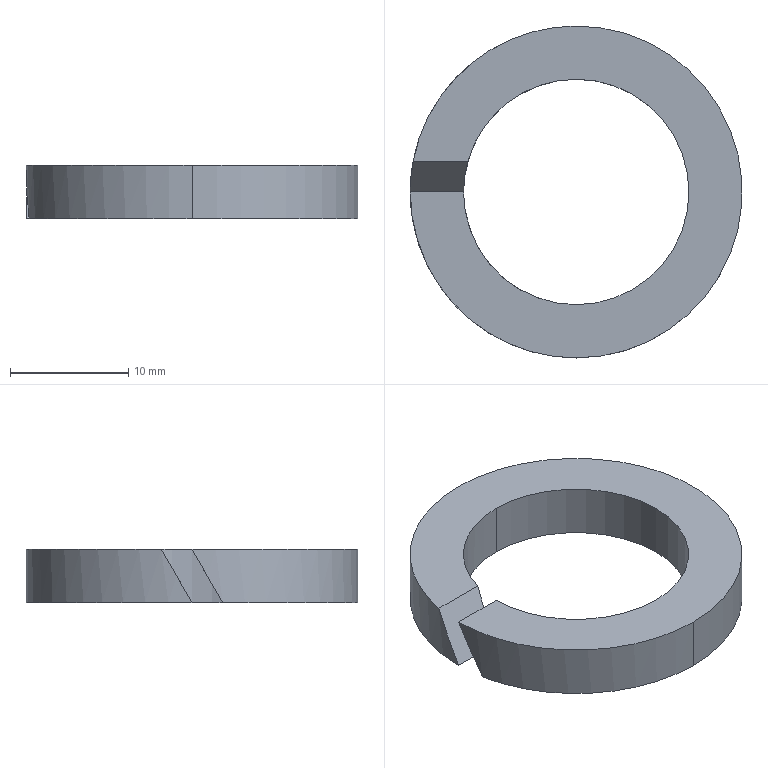Component | SolidWorks | Cylinder-1_spring lock washers--normal type gb-11 | 1 solid | 10 faces | box 28.04 x 28.04 x 4.5 mm | volume 1445 mm3 | cylinder 6 | plane 4 | commonest cylinder face diameters 19.04 x3 28.04 x3
build123d program:
from build123d import *

# Parameters (mm, degrees)
SKETCH1_R          = 14.02
SKETCH1_R_2        = 9.52
BASE_EXTRUDE_DEPTH = 4.5
CUT_EXTRUDE1_DEPTH = 21.332


with BuildPart() as part:
    # Sketch1 → Base-Extrude (new body)
    with BuildSketch(Plane.XY):
        Circle(SKETCH1_R)
        Circle(SKETCH1_R_2, mode=Mode.SUBTRACT)
    extrude(amount=-BASE_EXTRUDE_DEPTH)

    # Sketch2 → Cut-Extrude1 (cut, through all)
    with BuildSketch(Plane(origin=(0, 0, 0), x_dir=(1, 0, 0), z_dir=(0, 1, 0))):
        Polygon((0, 4.5), (2.598, 0), (0, 0), (-2.598, 4.5), align=None)
    extrude(amount=CUT_EXTRUDE1_DEPTH, mode=Mode.SUBTRACT)


solid = part.part

# Placed as in the assembly
solid = solid.moved(Location((-180.557, 26.412, -327.351), (0, 0, 90)))
STEP:
#1=COLOUR_RGB('',0.7922,0.8196,0.9333);
#2=FILL_AREA_STYLE_COLOUR('',#1);
#3=FILL_AREA_STYLE('',(#2));
#4=SURFACE_STYLE_FILL_AREA(#3);
#5=SURFACE_SIDE_STYLE('',(#4));
#6=SURFACE_STYLE_USAGE(.BOTH.,#5);
#7=PRESENTATION_STYLE_ASSIGNMENT((#6));
#8=CARTESIAN_POINT('',(-7.109,1.415,-12.888));
#9=VERTEX_POINT('',#8);
#10=CARTESIAN_POINT('',(-7.109,0.665,-12.888));
#11=VERTEX_POINT('',#10);
#12=CARTESIAN_POINT('',(-7.109,1.04,-12.888));
#13=DIRECTION('',(0.,-0.,-1.));
#14=DIRECTION('',(0.,-1.,0.));
#15=AXIS2_PLACEMENT_3D('',#12,#13,#14);
#16=CIRCLE('',#15,0.3748);
#17=EDGE_CURVE('',#9,#11,#16,.T.);
#18=ORIENTED_EDGE('',*,*,#17,.F.);
#19=CARTESIAN_POINT('',(-7.109,1.415,-13.065));
#20=VERTEX_POINT('',#19);
#21=CARTESIAN_POINT('',(-7.109,1.415,-12.888));
#22=DIRECTION('',(0.,-0.,-1.));
#23=VECTOR('',#22,39.37);
#24=LINE('',#21,#23);
#25=EDGE_CURVE('',#9,#20,#24,.T.);
#26=ORIENTED_EDGE('',*,*,#25,.T.);
#27=CARTESIAN_POINT('',(-7.109,0.665,-13.065));
#28=VERTEX_POINT('',#27);
#29=CARTESIAN_POINT('',(-7.109,1.04,-13.065));
#30=DIRECTION('',(0.,-0.,-1.));
#31=DIRECTION('',(0.,-1.,0.));
#32=AXIS2_PLACEMENT_3D('',#29,#30,#31);
#33=CIRCLE('',#32,0.3748);
#34=EDGE_CURVE('',#20,#28,#33,.T.);
#35=ORIENTED_EDGE('',*,*,#34,.T.);
#36=CARTESIAN_POINT('',(-7.109,0.665,-12.888));
#37=DIRECTION('',(0.,-0.,-1.));
#38=VECTOR('',#37,39.37);
#39=LINE('',#36,#38);
#40=EDGE_CURVE('',#11,#28,#39,.T.);
#41=ORIENTED_EDGE('',*,*,#40,.F.);
#42=EDGE_LOOP('',(#18,#26,#35,#41));
#43=FACE_OUTER_BOUND('',#42,.T.);
#44=CARTESIAN_POINT('',(-7.109,1.04,-12.888));
#45=DIRECTION('',(0.,-0.,-1.));
#46=DIRECTION('',(0.,-1.,0.));
#47=AXIS2_PLACEMENT_3D('',#44,#45,#46);
#48=CYLINDRICAL_SURFACE('',#47,0.3748);
#49=ADVANCED_FACE('',(#43),#48,.F.);
#50=CARTESIAN_POINT('',(-7.483,1.04,-12.888));
#51=VERTEX_POINT('',#50);
#52=CARTESIAN_POINT('',(-7.109,1.04,-12.888));
#53=DIRECTION('',(0.,-0.,-1.));
#54=DIRECTION('',(0.,-1.,0.));
#55=AXIS2_PLACEMENT_3D('',#52,#53,#54);
#56=CIRCLE('',#55,0.3748);
#57=EDGE_CURVE('',#11,#51,#56,.T.);
#58=ORIENTED_EDGE('',*,*,#57,.F.);
#59=ORIENTED_EDGE('',*,*,#40,.T.);
#60=CARTESIAN_POINT('',(-7.469,0.9376,-13.065));
#61=VERTEX_POINT('',#60);
#62=CARTESIAN_POINT('',(-7.109,1.04,-13.065));
#63=DIRECTION('',(0.,-0.,-1.));
#64=DIRECTION('',(0.,-1.,0.));
#65=AXIS2_PLACEMENT_3D('',#62,#63,#64);
#66=CIRCLE('',#65,0.3748);
#67=EDGE_CURVE('',#28,#61,#66,.T.);
#68=ORIENTED_EDGE('',*,*,#67,.T.);
#69=CARTESIAN_POINT('',(-7.483,1.04,-12.888));
#70=CARTESIAN_POINT('',(-7.483,1.005,-12.948));
#71=CARTESIAN_POINT('',(-7.479,0.9709,-13.007));
#72=CARTESIAN_POINT('',(-7.469,0.9376,-13.065));
#73=(BOUNDED_CURVE()B_SPLINE_CURVE(3,(#69,#70,#71,#72),.UNSPECIFIED.,.F.,.F.)B_SPLINE_CURVE_WITH_KNOTS((4,4),(4.712,4.989),.UNSPECIFIED.)CURVE()GEOMETRIC_REPRESENTATION_ITEM()RATIONAL_B_SPLINE_CURVE((1.,0.9936,0.9936,1.))REPRESENTATION_ITEM(''));
#74=EDGE_CURVE('',#51,#61,#73,.T.);
#75=ORIENTED_EDGE('',*,*,#74,.F.);
#76=EDGE_LOOP('',(#58,#59,#68,#75));
#77=FACE_OUTER_BOUND('',#76,.T.);
#78=CARTESIAN_POINT('',(-7.109,1.04,-12.888));
#79=DIRECTION('',(0.,-0.,-1.));
#80=DIRECTION('',(0.,-1.,0.));
#81=AXIS2_PLACEMENT_3D('',#78,#79,#80);
#82=CYLINDRICAL_SURFACE('',#81,0.3748);
#83=ADVANCED_FACE('',(#77),#82,.F.);
#84=CARTESIAN_POINT('',(-7.651,1.142,-12.888));
#85=VERTEX_POINT('',#84);
#86=CARTESIAN_POINT('',(-7.109,1.592,-12.888));
#87=VERTEX_POINT('',#86);
#88=CARTESIAN_POINT('',(-7.109,1.04,-12.888));
#89=DIRECTION('',(0.,-0.,-1.));
#90=DIRECTION('',(0.,-1.,0.));
#91=AXIS2_PLACEMENT_3D('',#88,#89,#90);
#92=CIRCLE('',#91,0.552);
#93=EDGE_CURVE('',#85,#87,#92,.T.);
#94=ORIENTED_EDGE('',*,*,#93,.T.);
#95=CARTESIAN_POINT('',(-7.109,1.592,-13.065));
#96=VERTEX_POINT('',#95);
#97=CARTESIAN_POINT('',(-7.109,1.592,-12.888));
#98=DIRECTION('',(0.,-0.,-1.));
#99=VECTOR('',#98,39.37);
#100=LINE('',#97,#99);
#101=EDGE_CURVE('',#87,#96,#100,.T.);
#102=ORIENTED_EDGE('',*,*,#101,.T.);
#103=CARTESIAN_POINT('',(-7.661,1.04,-13.065));
#104=VERTEX_POINT('',#103);
#105=CARTESIAN_POINT('',(-7.109,1.04,-13.065));
#106=DIRECTION('',(0.,-0.,-1.));
#107=DIRECTION('',(0.,-1.,0.));
#108=AXIS2_PLACEMENT_3D('',#105,#106,#107);
#109=CIRCLE('',#108,0.552);
#110=EDGE_CURVE('',#104,#96,#109,.T.);
#111=ORIENTED_EDGE('',*,*,#110,.F.);
#112=CARTESIAN_POINT('',(-7.661,1.04,-13.065));
#113=CARTESIAN_POINT('',(-7.661,1.074,-13.006));
#114=CARTESIAN_POINT('',(-7.657,1.108,-12.946));
#115=CARTESIAN_POINT('',(-7.651,1.142,-12.888));
#116=(BOUNDED_CURVE()B_SPLINE_CURVE(3,(#112,#113,#114,#115),.UNSPECIFIED.,.F.,.T.)B_SPLINE_CURVE_WITH_KNOTS((4,4),(1.571,1.757),.UNSPECIFIED.)CURVE()GEOMETRIC_REPRESENTATION_ITEM()RATIONAL_B_SPLINE_CURVE((1.,0.9971,0.9971,1.))REPRESENTATION_ITEM(''));
#117=EDGE_CURVE('',#104,#85,#116,.T.);
#118=ORIENTED_EDGE('',*,*,#117,.T.);
#119=EDGE_LOOP('',(#94,#102,#111,#118));
#120=FACE_OUTER_BOUND('',#119,.T.);
#121=CARTESIAN_POINT('',(-7.109,1.04,-12.888));
#122=DIRECTION('',(0.,-0.,-1.));
#123=DIRECTION('',(0.,-1.,0.));
#124=AXIS2_PLACEMENT_3D('',#121,#122,#123);
#125=CYLINDRICAL_SURFACE('',#124,0.552);
#126=ADVANCED_FACE('',(#120),#125,.T.);
#127=ORIENTED_EDGE('',*,*,#101,.F.);
#128=CARTESIAN_POINT('',(-7.109,0.4879,-12.888));
#129=VERTEX_POINT('',#128);
#130=CARTESIAN_POINT('',(-7.109,1.04,-12.888));
#131=DIRECTION('',(0.,-0.,-1.));
#132=DIRECTION('',(0.,-1.,0.));
#133=AXIS2_PLACEMENT_3D('',#130,#131,#132);
#134=CIRCLE('',#133,0.552);
#135=EDGE_CURVE('',#87,#129,#134,.T.);
#136=ORIENTED_EDGE('',*,*,#135,.T.);
#137=CARTESIAN_POINT('',(-7.109,0.4879,-13.065));
#138=VERTEX_POINT('',#137);
#139=CARTESIAN_POINT('',(-7.109,0.4879,-12.888));
#140=DIRECTION('',(0.,-0.,-1.));
#141=VECTOR('',#140,39.37);
#142=LINE('',#139,#141);
#143=EDGE_CURVE('',#129,#138,#142,.T.);
#144=ORIENTED_EDGE('',*,*,#143,.T.);
#145=CARTESIAN_POINT('',(-7.109,1.04,-13.065));
#146=DIRECTION('',(0.,-0.,-1.));
#147=DIRECTION('',(0.,-1.,0.));
#148=AXIS2_PLACEMENT_3D('',#145,#146,#147);
#149=CIRCLE('',#148,0.552);
#150=EDGE_CURVE('',#96,#138,#149,.T.);
#151=ORIENTED_EDGE('',*,*,#150,.F.);
#152=EDGE_LOOP('',(#127,#136,#144,#151));
#153=FACE_OUTER_BOUND('',#152,.T.);
#154=CARTESIAN_POINT('',(-7.109,1.04,-12.888));
#155=DIRECTION('',(0.,-0.,-1.));
#156=DIRECTION('',(0.,-1.,0.));
#157=AXIS2_PLACEMENT_3D('',#154,#155,#156);
#158=CYLINDRICAL_SURFACE('',#157,0.552);
#159=ADVANCED_FACE('',(#153),#158,.T.);
#160=ORIENTED_EDGE('',*,*,#143,.F.);
#161=CARTESIAN_POINT('',(-7.661,1.04,-12.888));
#162=VERTEX_POINT('',#161);
#163=CARTESIAN_POINT('',(-7.109,1.04,-12.888));
#164=DIRECTION('',(0.,-0.,-1.));
#165=DIRECTION('',(0.,-1.,0.));
#166=AXIS2_PLACEMENT_3D('',#163,#164,#165);
#167=CIRCLE('',#166,0.552);
#168=EDGE_CURVE('',#129,#162,#167,.T.);
#169=ORIENTED_EDGE('',*,*,#168,.T.);
#170=CARTESIAN_POINT('',(-7.651,0.9376,-13.065));
#171=VERTEX_POINT('',#170);
#172=CARTESIAN_POINT('',(-7.661,1.04,-12.888));
#173=CARTESIAN_POINT('',(-7.661,1.005,-12.947));
#174=CARTESIAN_POINT('',(-7.657,0.9713,-13.007));
#175=CARTESIAN_POINT('',(-7.651,0.9376,-13.065));
#176=(BOUNDED_CURVE()B_SPLINE_CURVE(3,(#172,#173,#174,#175),.UNSPECIFIED.,.F.,.F.)B_SPLINE_CURVE_WITH_KNOTS((4,4),(4.712,4.899),.UNSPECIFIED.)CURVE()GEOMETRIC_REPRESENTATION_ITEM()RATIONAL_B_SPLINE_CURVE((1.,0.9971,0.9971,1.))REPRESENTATION_ITEM(''));
#177=EDGE_CURVE('',#162,#171,#176,.T.);
#178=ORIENTED_EDGE('',*,*,#177,.T.);
#179=CARTESIAN_POINT('',(-7.109,1.04,-13.065));
#180=DIRECTION('',(0.,-0.,-1.));
#181=DIRECTION('',(0.,-1.,0.));
#182=AXIS2_PLACEMENT_3D('',#179,#180,#181);
#183=CIRCLE('',#182,0.552);
#184=EDGE_CURVE('',#138,#171,#183,.T.);
#185=ORIENTED_EDGE('',*,*,#184,.F.);
#186=EDGE_LOOP('',(#160,#169,#178,#185));
#187=FACE_OUTER_BOUND('',#186,.T.);
#188=CARTESIAN_POINT('',(-7.109,1.04,-12.888));
#189=DIRECTION('',(0.,-0.,-1.));
#190=DIRECTION('',(0.,-1.,0.));
#191=AXIS2_PLACEMENT_3D('',#188,#189,#190);
#192=CYLINDRICAL_SURFACE('',#191,0.552);
#193=ADVANCED_FACE('',(#187),#192,.T.);
#194=CARTESIAN_POINT('',(-7.469,1.142,-12.888));
#195=VERTEX_POINT('',#194);
#196=CARTESIAN_POINT('',(-7.661,1.142,-12.888));
#197=DIRECTION('',(1.,-0.,0.));
#198=VECTOR('',#197,39.37);
#199=LINE('',#196,#198);
#200=EDGE_CURVE('',#85,#195,#199,.T.);
#201=ORIENTED_EDGE('',*,*,#200,.T.);
#202=CARTESIAN_POINT('',(-7.109,1.04,-12.888));
#203=DIRECTION('',(0.,-0.,-1.));
#204=DIRECTION('',(0.,-1.,0.));
#205=AXIS2_PLACEMENT_3D('',#202,#203,#204);
#206=CIRCLE('',#205,0.3748);
#207=EDGE_CURVE('',#195,#9,#206,.T.);
#208=ORIENTED_EDGE('',*,*,#207,.T.);
#209=ORIENTED_EDGE('',*,*,#17,.T.);
#210=ORIENTED_EDGE('',*,*,#57,.T.);
#211=CARTESIAN_POINT('',(-7.661,1.04,-12.888));
#212=DIRECTION('',(1.,-0.,0.));
#213=VECTOR('',#212,39.37);
#214=LINE('',#211,#213);
#215=EDGE_CURVE('',#162,#51,#214,.T.);
#216=ORIENTED_EDGE('',*,*,#215,.F.);
#217=ORIENTED_EDGE('',*,*,#168,.F.);
#218=ORIENTED_EDGE('',*,*,#135,.F.);
#219=ORIENTED_EDGE('',*,*,#93,.F.);
#220=EDGE_LOOP('',(#201,#208,#209,#210,#216,#217,#218,#219));
#221=FACE_OUTER_BOUND('',#220,.T.);
#222=CARTESIAN_POINT('',(-7.109,1.04,-12.888));
#223=DIRECTION('',(0.,-0.,-1.));
#224=DIRECTION('',(-0.,-1.,0.));
#225=AXIS2_PLACEMENT_3D('',#222,#223,#224);
#226=PLANE('',#225);
#227=ADVANCED_FACE('',(#221),#226,.F.);
#228=CARTESIAN_POINT('',(-7.483,1.04,-13.065));
#229=VERTEX_POINT('',#228);
#230=CARTESIAN_POINT('',(-7.109,1.04,-13.065));
#231=DIRECTION('',(0.,-0.,-1.));
#232=DIRECTION('',(0.,-1.,0.));
#233=AXIS2_PLACEMENT_3D('',#230,#231,#232);
#234=CIRCLE('',#233,0.3748);
#235=EDGE_CURVE('',#229,#20,#234,.T.);
#236=ORIENTED_EDGE('',*,*,#235,.F.);
#237=CARTESIAN_POINT('',(-7.661,1.04,-13.065));
#238=DIRECTION('',(1.,-0.,0.));
#239=VECTOR('',#238,39.37);
#240=LINE('',#237,#239);
#241=EDGE_CURVE('',#104,#229,#240,.T.);
#242=ORIENTED_EDGE('',*,*,#241,.F.);
#243=ORIENTED_EDGE('',*,*,#110,.T.);
#244=ORIENTED_EDGE('',*,*,#150,.T.);
#245=ORIENTED_EDGE('',*,*,#184,.T.);
#246=CARTESIAN_POINT('',(-7.661,0.9376,-13.065));
#247=DIRECTION('',(1.,-0.,0.));
#248=VECTOR('',#247,39.37);
#249=LINE('',#246,#248);
#250=EDGE_CURVE('',#171,#61,#249,.T.);
#251=ORIENTED_EDGE('',*,*,#250,.T.);
#252=ORIENTED_EDGE('',*,*,#67,.F.);
#253=ORIENTED_EDGE('',*,*,#34,.F.);
#254=EDGE_LOOP('',(#236,#242,#243,#244,#245,#251,#252,#253));
#255=FACE_OUTER_BOUND('',#254,.T.);
#256=CARTESIAN_POINT('',(-7.109,1.04,-13.065));
#257=DIRECTION('',(0.,-0.,-1.));
#258=DIRECTION('',(-0.,-1.,0.));
#259=AXIS2_PLACEMENT_3D('',#256,#257,#258);
#260=PLANE('',#259);
#261=ADVANCED_FACE('',(#255),#260,.T.);
#262=ORIENTED_EDGE('',*,*,#25,.F.);
#263=ORIENTED_EDGE('',*,*,#207,.F.);
#264=CARTESIAN_POINT('',(-7.483,1.04,-13.065));
#265=CARTESIAN_POINT('',(-7.483,1.074,-13.005));
#266=CARTESIAN_POINT('',(-7.479,1.109,-12.946));
#267=CARTESIAN_POINT('',(-7.469,1.142,-12.888));
#268=(BOUNDED_CURVE()B_SPLINE_CURVE(3,(#264,#265,#266,#267),.UNSPECIFIED.,.F.,.F.)B_SPLINE_CURVE_WITH_KNOTS((4,4),(1.571,1.847),.UNSPECIFIED.)CURVE()GEOMETRIC_REPRESENTATION_ITEM()RATIONAL_B_SPLINE_CURVE((1.,0.9936,0.9936,1.))REPRESENTATION_ITEM(''));
#269=EDGE_CURVE('',#229,#195,#268,.T.);
#270=ORIENTED_EDGE('',*,*,#269,.F.);
#271=ORIENTED_EDGE('',*,*,#235,.T.);
#272=EDGE_LOOP('',(#262,#263,#270,#271));
#273=FACE_OUTER_BOUND('',#272,.T.);
#274=CARTESIAN_POINT('',(-7.109,1.04,-12.888));
#275=DIRECTION('',(0.,-0.,-1.));
#276=DIRECTION('',(0.,-1.,0.));
#277=AXIS2_PLACEMENT_3D('',#274,#275,#276);
#278=CYLINDRICAL_SURFACE('',#277,0.3748);
#279=ADVANCED_FACE('',(#273),#278,.F.);
#280=ORIENTED_EDGE('',*,*,#215,.T.);
#281=ORIENTED_EDGE('',*,*,#74,.T.);
#282=ORIENTED_EDGE('',*,*,#250,.F.);
#283=ORIENTED_EDGE('',*,*,#177,.F.);
#284=EDGE_LOOP('',(#280,#281,#282,#283));
#285=FACE_OUTER_BOUND('',#284,.T.);
#286=CARTESIAN_POINT('',(-7.661,1.04,-12.888));
#287=DIRECTION('',(0.,0.866,-0.5));
#288=DIRECTION('',(-0.,-0.5,-0.866));
#289=AXIS2_PLACEMENT_3D('',#286,#287,#288);
#290=PLANE('',#289);
#291=ADVANCED_FACE('',(#285),#290,.T.);
#292=ORIENTED_EDGE('',*,*,#241,.T.);
#293=ORIENTED_EDGE('',*,*,#269,.T.);
#294=ORIENTED_EDGE('',*,*,#200,.F.);
#295=ORIENTED_EDGE('',*,*,#117,.F.);
#296=EDGE_LOOP('',(#292,#293,#294,#295));
#297=FACE_OUTER_BOUND('',#296,.T.);
#298=CARTESIAN_POINT('',(-7.661,1.04,-13.065));
#299=DIRECTION('',(-0.,-0.866,0.5));
#300=DIRECTION('',(0.,0.5,0.866));
#301=AXIS2_PLACEMENT_3D('',#298,#299,#300);
#302=PLANE('',#301);
#303=ADVANCED_FACE('',(#297),#302,.T.);
#304=CLOSED_SHELL('',(#49,#83,#126,#159,#193,#227,#261,#279,#291,#303));
#305=MANIFOLD_SOLID_BREP('',#304);
#306=STYLED_ITEM('',(#7),#305);
#307=PRESENTATION_LAYER_ASSIGNMENT('','',(#306));
#308=CARTESIAN_POINT('',(0.,0.,0.));
#309=DIRECTION('',(0.,0.,1.));
#310=DIRECTION('',(1.,0.,0.));
#311=AXIS2_PLACEMENT_3D('',#308,#309,#310);
#312=(LENGTH_UNIT()NAMED_UNIT(*)SI_UNIT($,.METRE.));
#313=LENGTH_MEASURE_WITH_UNIT(LENGTH_MEASURE(0.0254),#312);
#314=DIMENSIONAL_EXPONENTS(1.,0.,0.,0.,0.,0.,0.);
#315=(CONVERSION_BASED_UNIT('',#313)LENGTH_UNIT()NAMED_UNIT(#314));
#316=UNCERTAINTY_MEASURE_WITH_UNIT(LENGTH_MEASURE(0.00001),#315,'','');
#317=(NAMED_UNIT(*)PLANE_ANGLE_UNIT()SI_UNIT($,.RADIAN.));
#318=(NAMED_UNIT(*)SI_UNIT($,.STERADIAN.)SOLID_ANGLE_UNIT());
#319=(GEOMETRIC_REPRESENTATION_CONTEXT(3)GLOBAL_UNCERTAINTY_ASSIGNED_CONTEXT((#316))GLOBAL_UNIT_ASSIGNED_CONTEXT((#315,#317,#318))REPRESENTATION_CONTEXT('',''));
#320=ADVANCED_BREP_SHAPE_REPRESENTATION('',(#305,#311),#319);
#321=(LENGTH_UNIT()NAMED_UNIT(*)SI_UNIT($,.METRE.));
#322=LENGTH_MEASURE_WITH_UNIT(LENGTH_MEASURE(0.0254),#321);
#323=DIMENSIONAL_EXPONENTS(1.,0.,0.,0.,0.,0.,0.);
#324=(CONVERSION_BASED_UNIT('',#322)LENGTH_UNIT()NAMED_UNIT(#323));
#325=UNCERTAINTY_MEASURE_WITH_UNIT(LENGTH_MEASURE(0.00001),#324,'','');
#326=(NAMED_UNIT(*)PLANE_ANGLE_UNIT()SI_UNIT($,.RADIAN.));
#327=(NAMED_UNIT(*)SI_UNIT($,.STERADIAN.)SOLID_ANGLE_UNIT());
#328=(GEOMETRIC_REPRESENTATION_CONTEXT(3)GLOBAL_UNCERTAINTY_ASSIGNED_CONTEXT((#325))GLOBAL_UNIT_ASSIGNED_CONTEXT((#324,#326,#327))REPRESENTATION_CONTEXT('',''));
#329=MECHANICAL_DESIGN_GEOMETRIC_PRESENTATION_REPRESENTATION('',(#306),#328);